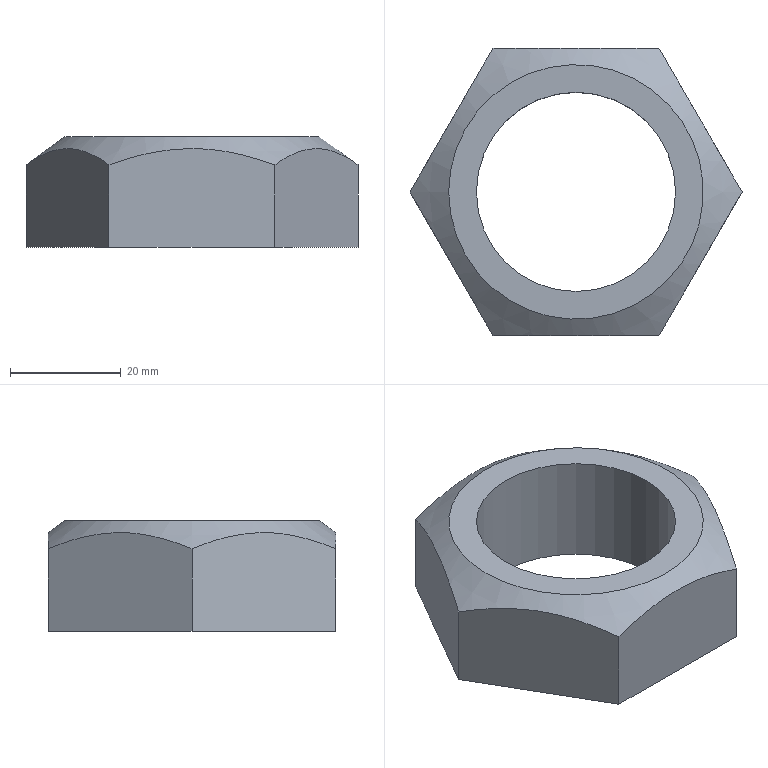Component | NX | A_PART_10 | 1 solid | 10 faces | box 60 x 51.96 x 20 mm | volume 25237 mm3 | plane 8 | cylinder 1 | cone 1 | commonest cylinder face diameters 36 x1
STEP:
#1=CARTESIAN_POINT('',(0.,0.,0.));
#2=DIRECTION('',(0.,0.,1.));
#3=DIRECTION('',(1.,0.,0.));
#4=AXIS2_PLACEMENT_3D('',#1,#2,#3);
#5=CARTESIAN_POINT('',(370.917,257.26,87.984));
#6=VERTEX_POINT('',#5);
#7=CARTESIAN_POINT('',(352.917,257.26,87.984));
#8=DIRECTION('',(0.,0.,1.));
#9=DIRECTION('',(1.,0.,0.));
#10=AXIS2_PLACEMENT_3D('',#7,#8,#9);
#11=CIRCLE('',#10,18.);
#12=CARTESIAN_POINT('',(352.917,257.26,87.984));
#13=DIRECTION('',(0.,0.,1.));
#14=DIRECTION('',(1.,0.,0.));
#15=AXIS2_PLACEMENT_3D('',#12,#13,#14);
#16=PLANE('',#15);
#17=CARTESIAN_POINT('',(0.,0.));
#18=DIRECTION('',(1.,0.));
#19=AXIS2_PLACEMENT_2D('',#17,#18);
#20=CIRCLE('',#19,18.);
#21=(GEOMETRIC_REPRESENTATION_CONTEXT(2)PARAMETRIC_REPRESENTATION_CONTEXT()REPRESENTATION_CONTEXT('',''));
#22=DEFINITIONAL_REPRESENTATION('',(#20),#21);
#23=PCURVE('',#16,#22);
#24=CARTESIAN_POINT('',(352.917,257.26,87.984));
#25=DIRECTION('',(0.,0.,-1.));
#26=DIRECTION('',(-1.,0.,0.));
#27=AXIS2_PLACEMENT_3D('',#24,#25,#26);
#28=CYLINDRICAL_SURFACE('',#27,18.);
#29=CARTESIAN_POINT('',(9.425,0.));
#30=DIRECTION('',(-1.,0.));
#31=VECTOR('',#30,1.);
#32=LINE('',#29,#31);
#33=(GEOMETRIC_REPRESENTATION_CONTEXT(2)PARAMETRIC_REPRESENTATION_CONTEXT()REPRESENTATION_CONTEXT('',''));
#34=DEFINITIONAL_REPRESENTATION('',(#32),#33);
#35=PCURVE('',#28,#34);
#36=SURFACE_CURVE('',#11,(#23,#35),.PCURVE_S1.);
#37=EDGE_CURVE('',#6,#6,#36,.T.);
#38=ORIENTED_EDGE('',*,*,#37,.F.);
#39=EDGE_LOOP('',(#38));
#40=FACE_BOUND('',#39,.T.);
#41=CARTESIAN_POINT('',(329.917,257.26,87.984));
#42=VERTEX_POINT('',#41);
#43=CARTESIAN_POINT('',(352.917,257.26,87.984));
#44=DIRECTION('',(0.,0.,-1.));
#45=DIRECTION('',(-1.,0.,0.));
#46=AXIS2_PLACEMENT_3D('',#43,#44,#45);
#47=CIRCLE('',#46,23.);
#48=CARTESIAN_POINT('',(-23.,0.));
#49=CARTESIAN_POINT('',(-23.,39.837));
#50=CARTESIAN_POINT('',(11.5,19.919));
#51=CARTESIAN_POINT('',(46.,0.));
#52=CARTESIAN_POINT('',(11.5,-19.919));
#53=CARTESIAN_POINT('',(-23.,-39.837));
#54=CARTESIAN_POINT('',(-23.,0.));
#55=(BOUNDED_CURVE()B_SPLINE_CURVE(2,(#48,#49,#50,#51,#52,#53,#54),.UNSPECIFIED.,.T.,.F.)B_SPLINE_CURVE_WITH_KNOTS((1,2,2,2,2,1),(-2.094,0.,2.094,4.189,6.283,8.378),.UNSPECIFIED.)CURVE()GEOMETRIC_REPRESENTATION_ITEM()RATIONAL_B_SPLINE_CURVE((1.,0.5,1.,0.5,1.,0.5,1.))REPRESENTATION_ITEM(''));
#56=(GEOMETRIC_REPRESENTATION_CONTEXT(2)PARAMETRIC_REPRESENTATION_CONTEXT()REPRESENTATION_CONTEXT('',''));
#57=DEFINITIONAL_REPRESENTATION('',(#55),#56);
#58=PCURVE('',#16,#57);
#59=CARTESIAN_POINT('',(352.917,257.26,87.984));
#60=DIRECTION('',(0.,0.,-1.));
#61=DIRECTION('',(-1.,0.,0.));
#62=AXIS2_PLACEMENT_3D('',#59,#60,#61);
#63=CONICAL_SURFACE('',#62,23.,0.9425);
#64=CARTESIAN_POINT('',(0.,0.));
#65=DIRECTION('',(1.,0.));
#66=VECTOR('',#65,1.);
#67=LINE('',#64,#66);
#68=(GEOMETRIC_REPRESENTATION_CONTEXT(2)PARAMETRIC_REPRESENTATION_CONTEXT()REPRESENTATION_CONTEXT('',''));
#69=DEFINITIONAL_REPRESENTATION('',(#67),#68);
#70=PCURVE('',#63,#69);
#71=SURFACE_CURVE('',#47,(#58,#70),.PCURVE_S1.);
#72=EDGE_CURVE('',#42,#42,#71,.T.);
#73=ORIENTED_EDGE('',*,*,#72,.F.);
#74=EDGE_LOOP('',(#73));
#75=FACE_BOUND('',#74,.T.);
#76=ADVANCED_FACE('',(#40,#75),#16,.T.);
#77=CARTESIAN_POINT('',(367.917,231.279,82.898));
#78=VERTEX_POINT('',#77);
#79=CARTESIAN_POINT('',(367.917,231.279,67.984));
#80=VERTEX_POINT('',#79);
#81=CARTESIAN_POINT('',(367.917,231.279,87.984));
#82=DIRECTION('',(0.,0.,-1.));
#83=VECTOR('',#82,1.);
#84=LINE('',#81,#83);
#85=CARTESIAN_POINT('',(337.917,231.279,87.984));
#86=DIRECTION('',(0.,1.,0.));
#87=DIRECTION('',(-1.,0.,0.));
#88=AXIS2_PLACEMENT_3D('',#85,#86,#87);
#89=PLANE('',#88);
#90=CARTESIAN_POINT('',(-30.,0.));
#91=DIRECTION('',(0.,-1.));
#92=VECTOR('',#91,1.);
#93=LINE('',#90,#92);
#94=(GEOMETRIC_REPRESENTATION_CONTEXT(2)PARAMETRIC_REPRESENTATION_CONTEXT()REPRESENTATION_CONTEXT('',''));
#95=DEFINITIONAL_REPRESENTATION('',(#93),#94);
#96=PCURVE('',#89,#95);
#97=CARTESIAN_POINT('',(367.917,231.279,87.984));
#98=DIRECTION('',(-0.866,0.5,0.));
#99=DIRECTION('',(-0.5,-0.866,0.));
#100=AXIS2_PLACEMENT_3D('',#97,#98,#99);
#101=PLANE('',#100);
#102=CARTESIAN_POINT('',(0.,0.));
#103=DIRECTION('',(0.,-1.));
#104=VECTOR('',#103,1.);
#105=LINE('',#102,#104);
#106=(GEOMETRIC_REPRESENTATION_CONTEXT(2)PARAMETRIC_REPRESENTATION_CONTEXT()REPRESENTATION_CONTEXT('',''));
#107=DEFINITIONAL_REPRESENTATION('',(#105),#106);
#108=PCURVE('',#101,#107);
#109=SURFACE_CURVE('',#84,(#96,#108),.PCURVE_S1.);
#110=EDGE_CURVE('',#78,#80,#109,.T.);
#111=ORIENTED_EDGE('',*,*,#110,.F.);
#112=CARTESIAN_POINT('',(337.917,231.279,82.898));
#113=VERTEX_POINT('',#112);
#114=CARTESIAN_POINT('',(367.917,231.279,82.898));
#115=CARTESIAN_POINT('',(365.498,231.279,83.776));
#116=CARTESIAN_POINT('',(363.045,231.279,84.51));
#117=CARTESIAN_POINT('',(358.03,231.279,85.536));
#118=CARTESIAN_POINT('',(355.435,231.279,85.821));
#119=CARTESIAN_POINT('',(347.77,231.279,85.813));
#120=CARTESIAN_POINT('',(342.723,231.279,84.644));
#121=CARTESIAN_POINT('',(337.917,231.279,82.898));
#122=B_SPLINE_CURVE_WITH_KNOTS('',3,(#114,#115,#116,#117,#118,#119,#120,#121),.UNSPECIFIED.,.F.,.F.,(4,2,2,4),(0.,0.25,0.5,1.),.UNSPECIFIED.);
#123=CARTESIAN_POINT('',(-30.,-5.086));
#124=CARTESIAN_POINT('',(-27.582,-4.207));
#125=CARTESIAN_POINT('',(-25.128,-3.474));
#126=CARTESIAN_POINT('',(-20.113,-2.448));
#127=CARTESIAN_POINT('',(-17.519,-2.163));
#128=CARTESIAN_POINT('',(-9.854,-2.171));
#129=CARTESIAN_POINT('',(-4.807,-3.34));
#130=CARTESIAN_POINT('',(0.,-5.086));
#131=B_SPLINE_CURVE_WITH_KNOTS('',3,(#123,#124,#125,#126,#127,#128,#129,#130),.UNSPECIFIED.,.F.,.F.,(4,2,2,4),(0.,0.25,0.5,1.),.UNSPECIFIED.);
#132=(GEOMETRIC_REPRESENTATION_CONTEXT(2)PARAMETRIC_REPRESENTATION_CONTEXT()REPRESENTATION_CONTEXT('',''));
#133=DEFINITIONAL_REPRESENTATION('',(#131),#132);
#134=PCURVE('',#89,#133);
#135=CARTESIAN_POINT('',(4.189,5.086));
#136=CARTESIAN_POINT('',(4.201,4.926));
#137=CARTESIAN_POINT('',(4.227,4.616));
#138=CARTESIAN_POINT('',(4.268,4.183));
#139=CARTESIAN_POINT('',(4.311,3.784));
#140=CARTESIAN_POINT('',(4.356,3.422));
#141=CARTESIAN_POINT('',(4.403,3.099));
#142=CARTESIAN_POINT('',(4.451,2.819));
#143=CARTESIAN_POINT('',(4.502,2.584));
#144=CARTESIAN_POINT('',(4.553,2.398));
#145=CARTESIAN_POINT('',(4.606,2.264));
#146=CARTESIAN_POINT('',(4.66,2.183));
#147=CARTESIAN_POINT('',(4.714,2.156));
#148=CARTESIAN_POINT('',(4.767,2.186));
#149=CARTESIAN_POINT('',(4.821,2.269));
#150=CARTESIAN_POINT('',(4.873,2.405));
#151=CARTESIAN_POINT('',(4.924,2.591));
#152=CARTESIAN_POINT('',(4.974,2.825));
#153=CARTESIAN_POINT('',(5.022,3.105));
#154=CARTESIAN_POINT('',(5.069,3.427));
#155=CARTESIAN_POINT('',(5.114,3.788));
#156=CARTESIAN_POINT('',(5.157,4.187));
#157=CARTESIAN_POINT('',(5.197,4.619));
#158=CARTESIAN_POINT('',(5.223,4.927));
#159=CARTESIAN_POINT('',(5.236,5.086));
#160=B_SPLINE_CURVE_WITH_KNOTS('',3,(#135,#136,#137,#138,#139,#140,#141,#142,#143,#144,#145,#146,#147,#148,#149,#150,#151,#152,#153,#154,#155,#156,#157,#158,#159),.UNSPECIFIED.,.F.,.F.,(4,1,1,1,1,1,1,1,1,1,1,1,1,1,1,1,1,1,1,1,1,1,4),(0.,0.04545,0.09091,0.1364,0.1818,0.2273,0.2727,0.3182,0.3636,0.4091,0.4545,0.5,0.5455,0.5909,0.6364,0.6818,0.7273,0.7727,0.8182,0.8636,0.9091,0.9545,1.),.QUASI_UNIFORM_KNOTS.);
#161=(GEOMETRIC_REPRESENTATION_CONTEXT(2)PARAMETRIC_REPRESENTATION_CONTEXT()REPRESENTATION_CONTEXT('',''));
#162=DEFINITIONAL_REPRESENTATION('',(#160),#161);
#163=PCURVE('',#63,#162);
#164=SURFACE_CURVE('',#122,(#134,#163),.PCURVE_S1.);
#165=EDGE_CURVE('',#78,#113,#164,.T.);
#166=ORIENTED_EDGE('',*,*,#165,.T.);
#167=CARTESIAN_POINT('',(337.917,231.279,67.984));
#168=VERTEX_POINT('',#167);
#169=CARTESIAN_POINT('',(337.917,231.279,87.984));
#170=DIRECTION('',(0.,0.,-1.));
#171=VECTOR('',#170,1.);
#172=LINE('',#169,#171);
#173=CARTESIAN_POINT('',(0.,0.));
#174=DIRECTION('',(0.,-1.));
#175=VECTOR('',#174,1.);
#176=LINE('',#173,#175);
#177=(GEOMETRIC_REPRESENTATION_CONTEXT(2)PARAMETRIC_REPRESENTATION_CONTEXT()REPRESENTATION_CONTEXT('',''));
#178=DEFINITIONAL_REPRESENTATION('',(#176),#177);
#179=PCURVE('',#89,#178);
#180=CARTESIAN_POINT('',(322.917,257.26,87.984));
#181=DIRECTION('',(0.866,0.5,0.));
#182=DIRECTION('',(-0.5,0.866,0.));
#183=AXIS2_PLACEMENT_3D('',#180,#181,#182);
#184=PLANE('',#183);
#185=CARTESIAN_POINT('',(-30.,0.));
#186=DIRECTION('',(0.,-1.));
#187=VECTOR('',#186,1.);
#188=LINE('',#185,#187);
#189=(GEOMETRIC_REPRESENTATION_CONTEXT(2)PARAMETRIC_REPRESENTATION_CONTEXT()REPRESENTATION_CONTEXT('',''));
#190=DEFINITIONAL_REPRESENTATION('',(#188),#189);
#191=PCURVE('',#184,#190);
#192=SURFACE_CURVE('',#172,(#179,#191),.PCURVE_S1.);
#193=EDGE_CURVE('',#113,#168,#192,.T.);
#194=ORIENTED_EDGE('',*,*,#193,.T.);
#195=CARTESIAN_POINT('',(337.917,231.279,67.984));
#196=DIRECTION('',(1.,-0.,0.));
#197=VECTOR('',#196,1.);
#198=LINE('',#195,#197);
#199=CARTESIAN_POINT('',(0.,-20.));
#200=DIRECTION('',(-1.,0.));
#201=VECTOR('',#200,1.);
#202=LINE('',#199,#201);
#203=(GEOMETRIC_REPRESENTATION_CONTEXT(2)PARAMETRIC_REPRESENTATION_CONTEXT()REPRESENTATION_CONTEXT('',''));
#204=DEFINITIONAL_REPRESENTATION('',(#202),#203);
#205=PCURVE('',#89,#204);
#206=CARTESIAN_POINT('',(352.917,257.26,67.984));
#207=DIRECTION('',(0.,0.,1.));
#208=DIRECTION('',(1.,0.,0.));
#209=AXIS2_PLACEMENT_3D('',#206,#207,#208);
#210=PLANE('',#209);
#211=CARTESIAN_POINT('',(-15.,-25.981));
#212=DIRECTION('',(1.,-0.));
#213=VECTOR('',#212,1.);
#214=LINE('',#211,#213);
#215=(GEOMETRIC_REPRESENTATION_CONTEXT(2)PARAMETRIC_REPRESENTATION_CONTEXT()REPRESENTATION_CONTEXT('',''));
#216=DEFINITIONAL_REPRESENTATION('',(#214),#215);
#217=PCURVE('',#210,#216);
#218=SURFACE_CURVE('',#198,(#205,#217),.PCURVE_S1.);
#219=EDGE_CURVE('',#168,#80,#218,.T.);
#220=ORIENTED_EDGE('',*,*,#219,.T.);
#221=EDGE_LOOP('',(#111,#166,#194,#220));
#222=FACE_BOUND('',#221,.T.);
#223=ADVANCED_FACE('',(#222),#89,.F.);
#224=CARTESIAN_POINT('',(382.917,257.26,82.898));
#225=VERTEX_POINT('',#224);
#226=CARTESIAN_POINT('',(382.917,257.26,67.984));
#227=VERTEX_POINT('',#226);
#228=CARTESIAN_POINT('',(382.917,257.26,87.984));
#229=DIRECTION('',(0.,0.,-1.));
#230=VECTOR('',#229,1.);
#231=LINE('',#228,#230);
#232=CARTESIAN_POINT('',(-30.,0.));
#233=DIRECTION('',(0.,-1.));
#234=VECTOR('',#233,1.);
#235=LINE('',#232,#234);
#236=(GEOMETRIC_REPRESENTATION_CONTEXT(2)PARAMETRIC_REPRESENTATION_CONTEXT()REPRESENTATION_CONTEXT('',''));
#237=DEFINITIONAL_REPRESENTATION('',(#235),#236);
#238=PCURVE('',#101,#237);
#239=CARTESIAN_POINT('',(382.917,257.26,87.984));
#240=DIRECTION('',(-0.866,-0.5,0.));
#241=DIRECTION('',(0.5,-0.866,0.));
#242=AXIS2_PLACEMENT_3D('',#239,#240,#241);
#243=PLANE('',#242);
#244=CARTESIAN_POINT('',(0.,0.));
#245=DIRECTION('',(0.,-1.));
#246=VECTOR('',#245,1.);
#247=LINE('',#244,#246);
#248=(GEOMETRIC_REPRESENTATION_CONTEXT(2)PARAMETRIC_REPRESENTATION_CONTEXT()REPRESENTATION_CONTEXT('',''));
#249=DEFINITIONAL_REPRESENTATION('',(#247),#248);
#250=PCURVE('',#243,#249);
#251=SURFACE_CURVE('',#231,(#238,#250),.PCURVE_S1.);
#252=EDGE_CURVE('',#225,#227,#251,.T.);
#253=ORIENTED_EDGE('',*,*,#252,.F.);
#254=CARTESIAN_POINT('',(382.917,257.26,82.898));
#255=CARTESIAN_POINT('',(380.496,253.067,84.657));
#256=CARTESIAN_POINT('',(378.023,248.783,85.808));
#257=CARTESIAN_POINT('',(374.164,242.099,85.823));
#258=CARTESIAN_POINT('',(372.869,239.857,85.538));
#259=CARTESIAN_POINT('',(370.361,235.513,84.515));
#260=CARTESIAN_POINT('',(369.131,233.382,83.78));
#261=CARTESIAN_POINT('',(367.917,231.279,82.898));
#262=B_SPLINE_CURVE_WITH_KNOTS('',3,(#254,#255,#256,#257,#258,#259,#260,#261),.UNSPECIFIED.,.F.,.F.,(4,2,2,4),(0.,0.5,0.75,1.),.UNSPECIFIED.);
#263=CARTESIAN_POINT('',(-30.,-5.086));
#264=CARTESIAN_POINT('',(-25.159,-3.327));
#265=CARTESIAN_POINT('',(-20.212,-2.175));
#266=CARTESIAN_POINT('',(-12.494,-2.161));
#267=CARTESIAN_POINT('',(-9.905,-2.445));
#268=CARTESIAN_POINT('',(-4.889,-3.469));
#269=CARTESIAN_POINT('',(-2.429,-4.204));
#270=CARTESIAN_POINT('',(0.,-5.086));
#271=B_SPLINE_CURVE_WITH_KNOTS('',3,(#263,#264,#265,#266,#267,#268,#269,#270),.UNSPECIFIED.,.F.,.F.,(4,2,2,4),(0.,0.5,0.75,1.),.UNSPECIFIED.);
#272=(GEOMETRIC_REPRESENTATION_CONTEXT(2)PARAMETRIC_REPRESENTATION_CONTEXT()REPRESENTATION_CONTEXT('',''));
#273=DEFINITIONAL_REPRESENTATION('',(#271),#272);
#274=PCURVE('',#101,#273);
#275=CARTESIAN_POINT('',(3.142,5.086));
#276=CARTESIAN_POINT('',(3.154,4.926));
#277=CARTESIAN_POINT('',(3.18,4.616));
#278=CARTESIAN_POINT('',(3.221,4.184));
#279=CARTESIAN_POINT('',(3.264,3.786));
#280=CARTESIAN_POINT('',(3.309,3.426));
#281=CARTESIAN_POINT('',(3.355,3.105));
#282=CARTESIAN_POINT('',(3.403,2.827));
#283=CARTESIAN_POINT('',(3.452,2.593));
#284=CARTESIAN_POINT('',(3.503,2.407));
#285=CARTESIAN_POINT('',(3.556,2.271));
#286=CARTESIAN_POINT('',(3.609,2.187));
#287=CARTESIAN_POINT('',(3.663,2.156));
#288=CARTESIAN_POINT('',(3.717,2.182));
#289=CARTESIAN_POINT('',(3.77,2.262));
#290=CARTESIAN_POINT('',(3.823,2.396));
#291=CARTESIAN_POINT('',(3.875,2.582));
#292=CARTESIAN_POINT('',(3.926,2.816));
#293=CARTESIAN_POINT('',(3.974,3.095));
#294=CARTESIAN_POINT('',(4.021,3.418));
#295=CARTESIAN_POINT('',(4.066,3.78));
#296=CARTESIAN_POINT('',(4.109,4.18));
#297=CARTESIAN_POINT('',(4.15,4.614));
#298=CARTESIAN_POINT('',(4.176,4.925));
#299=CARTESIAN_POINT('',(4.189,5.086));
#300=B_SPLINE_CURVE_WITH_KNOTS('',3,(#275,#276,#277,#278,#279,#280,#281,#282,#283,#284,#285,#286,#287,#288,#289,#290,#291,#292,#293,#294,#295,#296,#297,#298,#299),.UNSPECIFIED.,.F.,.F.,(4,1,1,1,1,1,1,1,1,1,1,1,1,1,1,1,1,1,1,1,1,1,4),(0.,0.04545,0.09091,0.1364,0.1818,0.2273,0.2727,0.3182,0.3636,0.4091,0.4545,0.5,0.5455,0.5909,0.6364,0.6818,0.7273,0.7727,0.8182,0.8636,0.9091,0.9545,1.),.QUASI_UNIFORM_KNOTS.);
#301=(GEOMETRIC_REPRESENTATION_CONTEXT(2)PARAMETRIC_REPRESENTATION_CONTEXT()REPRESENTATION_CONTEXT('',''));
#302=DEFINITIONAL_REPRESENTATION('',(#300),#301);
#303=PCURVE('',#63,#302);
#304=SURFACE_CURVE('',#262,(#274,#303),.PCURVE_S1.);
#305=EDGE_CURVE('',#225,#78,#304,.T.);
#306=ORIENTED_EDGE('',*,*,#305,.T.);
#307=ORIENTED_EDGE('',*,*,#110,.T.);
#308=CARTESIAN_POINT('',(367.917,231.279,67.984));
#309=DIRECTION('',(0.5,0.866,0.));
#310=VECTOR('',#309,1.);
#311=LINE('',#308,#310);
#312=CARTESIAN_POINT('',(0.,-20.));
#313=DIRECTION('',(-1.,0.));
#314=VECTOR('',#313,1.);
#315=LINE('',#312,#314);
#316=(GEOMETRIC_REPRESENTATION_CONTEXT(2)PARAMETRIC_REPRESENTATION_CONTEXT()REPRESENTATION_CONTEXT('',''));
#317=DEFINITIONAL_REPRESENTATION('',(#315),#316);
#318=PCURVE('',#101,#317);
#319=CARTESIAN_POINT('',(15.,-25.981));
#320=DIRECTION('',(0.5,0.866));
#321=VECTOR('',#320,1.);
#322=LINE('',#319,#321);
#323=(GEOMETRIC_REPRESENTATION_CONTEXT(2)PARAMETRIC_REPRESENTATION_CONTEXT()REPRESENTATION_CONTEXT('',''));
#324=DEFINITIONAL_REPRESENTATION('',(#322),#323);
#325=PCURVE('',#210,#324);
#326=SURFACE_CURVE('',#311,(#318,#325),.PCURVE_S1.);
#327=EDGE_CURVE('',#80,#227,#326,.T.);
#328=ORIENTED_EDGE('',*,*,#327,.T.);
#329=EDGE_LOOP('',(#253,#306,#307,#328));
#330=FACE_BOUND('',#329,.T.);
#331=ADVANCED_FACE('',(#330),#101,.F.);
#332=CARTESIAN_POINT('',(367.917,283.24,82.898));
#333=VERTEX_POINT('',#332);
#334=CARTESIAN_POINT('',(367.917,283.24,67.984));
#335=VERTEX_POINT('',#334);
#336=CARTESIAN_POINT('',(367.917,283.24,87.984));
#337=DIRECTION('',(0.,0.,-1.));
#338=VECTOR('',#337,1.);
#339=LINE('',#336,#338);
#340=CARTESIAN_POINT('',(-30.,0.));
#341=DIRECTION('',(0.,-1.));
#342=VECTOR('',#341,1.);
#343=LINE('',#340,#342);
#344=(GEOMETRIC_REPRESENTATION_CONTEXT(2)PARAMETRIC_REPRESENTATION_CONTEXT()REPRESENTATION_CONTEXT('',''));
#345=DEFINITIONAL_REPRESENTATION('',(#343),#344);
#346=PCURVE('',#243,#345);
#347=CARTESIAN_POINT('',(367.917,283.24,87.984));
#348=DIRECTION('',(-0.,-1.,0.));
#349=DIRECTION('',(1.,-0.,0.));
#350=AXIS2_PLACEMENT_3D('',#347,#348,#349);
#351=PLANE('',#350);
#352=CARTESIAN_POINT('',(0.,0.));
#353=DIRECTION('',(0.,-1.));
#354=VECTOR('',#353,1.);
#355=LINE('',#352,#354);
#356=(GEOMETRIC_REPRESENTATION_CONTEXT(2)PARAMETRIC_REPRESENTATION_CONTEXT()REPRESENTATION_CONTEXT('',''));
#357=DEFINITIONAL_REPRESENTATION('',(#355),#356);
#358=PCURVE('',#351,#357);
#359=SURFACE_CURVE('',#339,(#346,#358),.PCURVE_S1.);
#360=EDGE_CURVE('',#333,#335,#359,.T.);
#361=ORIENTED_EDGE('',*,*,#360,.F.);
#362=CARTESIAN_POINT('',(367.917,283.24,82.898));
#363=CARTESIAN_POINT('',(370.337,279.048,84.657));
#364=CARTESIAN_POINT('',(372.811,274.764,85.808));
#365=CARTESIAN_POINT('',(376.67,268.08,85.823));
#366=CARTESIAN_POINT('',(377.964,265.838,85.538));
#367=CARTESIAN_POINT('',(380.472,261.494,84.515));
#368=CARTESIAN_POINT('',(381.703,259.363,83.78));
#369=CARTESIAN_POINT('',(382.917,257.26,82.898));
#370=B_SPLINE_CURVE_WITH_KNOTS('',3,(#362,#363,#364,#365,#366,#367,#368,#369),.UNSPECIFIED.,.F.,.F.,(4,2,2,4),(0.,0.5,0.75,1.),.UNSPECIFIED.);
#371=CARTESIAN_POINT('',(-30.,-5.086));
#372=CARTESIAN_POINT('',(-25.159,-3.327));
#373=CARTESIAN_POINT('',(-20.212,-2.175));
#374=CARTESIAN_POINT('',(-12.494,-2.161));
#375=CARTESIAN_POINT('',(-9.905,-2.445));
#376=CARTESIAN_POINT('',(-4.889,-3.469));
#377=CARTESIAN_POINT('',(-2.429,-4.204));
#378=CARTESIAN_POINT('',(0.,-5.086));
#379=B_SPLINE_CURVE_WITH_KNOTS('',3,(#371,#372,#373,#374,#375,#376,#377,#378),.UNSPECIFIED.,.F.,.F.,(4,2,2,4),(0.,0.5,0.75,1.),.UNSPECIFIED.);
#380=(GEOMETRIC_REPRESENTATION_CONTEXT(2)PARAMETRIC_REPRESENTATION_CONTEXT()REPRESENTATION_CONTEXT('',''));
#381=DEFINITIONAL_REPRESENTATION('',(#379),#380);
#382=PCURVE('',#243,#381);
#383=CARTESIAN_POINT('',(2.094,5.086));
#384=CARTESIAN_POINT('',(2.107,4.926));
#385=CARTESIAN_POINT('',(2.133,4.616));
#386=CARTESIAN_POINT('',(2.174,4.184));
#387=CARTESIAN_POINT('',(2.217,3.786));
#388=CARTESIAN_POINT('',(2.261,3.426));
#389=CARTESIAN_POINT('',(2.308,3.105));
#390=CARTESIAN_POINT('',(2.356,2.827));
#391=CARTESIAN_POINT('',(2.405,2.593));
#392=CARTESIAN_POINT('',(2.456,2.407));
#393=CARTESIAN_POINT('',(2.508,2.271));
#394=CARTESIAN_POINT('',(2.562,2.187));
#395=CARTESIAN_POINT('',(2.615,2.156));
#396=CARTESIAN_POINT('',(2.669,2.182));
#397=CARTESIAN_POINT('',(2.723,2.262));
#398=CARTESIAN_POINT('',(2.776,2.396));
#399=CARTESIAN_POINT('',(2.828,2.582));
#400=CARTESIAN_POINT('',(2.878,2.816));
#401=CARTESIAN_POINT('',(2.927,3.095));
#402=CARTESIAN_POINT('',(2.974,3.418));
#403=CARTESIAN_POINT('',(3.019,3.78));
#404=CARTESIAN_POINT('',(3.062,4.18));
#405=CARTESIAN_POINT('',(3.103,4.614));
#406=CARTESIAN_POINT('',(3.129,4.925));
#407=CARTESIAN_POINT('',(3.142,5.086));
#408=B_SPLINE_CURVE_WITH_KNOTS('',3,(#383,#384,#385,#386,#387,#388,#389,#390,#391,#392,#393,#394,#395,#396,#397,#398,#399,#400,#401,#402,#403,#404,#405,#406,#407),.UNSPECIFIED.,.F.,.F.,(4,1,1,1,1,1,1,1,1,1,1,1,1,1,1,1,1,1,1,1,1,1,4),(0.,0.04545,0.09091,0.1364,0.1818,0.2273,0.2727,0.3182,0.3636,0.4091,0.4545,0.5,0.5455,0.5909,0.6364,0.6818,0.7273,0.7727,0.8182,0.8636,0.9091,0.9545,1.),.QUASI_UNIFORM_KNOTS.);
#409=(GEOMETRIC_REPRESENTATION_CONTEXT(2)PARAMETRIC_REPRESENTATION_CONTEXT()REPRESENTATION_CONTEXT('',''));
#410=DEFINITIONAL_REPRESENTATION('',(#408),#409);
#411=PCURVE('',#63,#410);
#412=SURFACE_CURVE('',#370,(#382,#411),.PCURVE_S1.);
#413=EDGE_CURVE('',#333,#225,#412,.T.);
#414=ORIENTED_EDGE('',*,*,#413,.T.);
#415=ORIENTED_EDGE('',*,*,#252,.T.);
#416=CARTESIAN_POINT('',(382.917,257.26,67.984));
#417=DIRECTION('',(-0.5,0.866,0.));
#418=VECTOR('',#417,1.);
#419=LINE('',#416,#418);
#420=CARTESIAN_POINT('',(0.,-20.));
#421=DIRECTION('',(-1.,0.));
#422=VECTOR('',#421,1.);
#423=LINE('',#420,#422);
#424=(GEOMETRIC_REPRESENTATION_CONTEXT(2)PARAMETRIC_REPRESENTATION_CONTEXT()REPRESENTATION_CONTEXT('',''));
#425=DEFINITIONAL_REPRESENTATION('',(#423),#424);
#426=PCURVE('',#243,#425);
#427=CARTESIAN_POINT('',(30.,0.));
#428=DIRECTION('',(-0.5,0.866));
#429=VECTOR('',#428,1.);
#430=LINE('',#427,#429);
#431=(GEOMETRIC_REPRESENTATION_CONTEXT(2)PARAMETRIC_REPRESENTATION_CONTEXT()REPRESENTATION_CONTEXT('',''));
#432=DEFINITIONAL_REPRESENTATION('',(#430),#431);
#433=PCURVE('',#210,#432);
#434=SURFACE_CURVE('',#419,(#426,#433),.PCURVE_S1.);
#435=EDGE_CURVE('',#227,#335,#434,.T.);
#436=ORIENTED_EDGE('',*,*,#435,.T.);
#437=EDGE_LOOP('',(#361,#414,#415,#436));
#438=FACE_BOUND('',#437,.T.);
#439=ADVANCED_FACE('',(#438),#243,.F.);
#440=CARTESIAN_POINT('',(337.917,283.24,82.898));
#441=VERTEX_POINT('',#440);
#442=CARTESIAN_POINT('',(337.917,283.24,67.984));
#443=VERTEX_POINT('',#442);
#444=CARTESIAN_POINT('',(337.917,283.24,87.984));
#445=DIRECTION('',(0.,0.,-1.));
#446=VECTOR('',#445,1.);
#447=LINE('',#444,#446);
#448=CARTESIAN_POINT('',(-30.,0.));
#449=DIRECTION('',(0.,-1.));
#450=VECTOR('',#449,1.);
#451=LINE('',#448,#450);
#452=(GEOMETRIC_REPRESENTATION_CONTEXT(2)PARAMETRIC_REPRESENTATION_CONTEXT()REPRESENTATION_CONTEXT('',''));
#453=DEFINITIONAL_REPRESENTATION('',(#451),#452);
#454=PCURVE('',#351,#453);
#455=CARTESIAN_POINT('',(337.917,283.24,87.984));
#456=DIRECTION('',(0.866,-0.5,0.));
#457=DIRECTION('',(0.5,0.866,0.));
#458=AXIS2_PLACEMENT_3D('',#455,#456,#457);
#459=PLANE('',#458);
#460=CARTESIAN_POINT('',(0.,0.));
#461=DIRECTION('',(0.,-1.));
#462=VECTOR('',#461,1.);
#463=LINE('',#460,#462);
#464=(GEOMETRIC_REPRESENTATION_CONTEXT(2)PARAMETRIC_REPRESENTATION_CONTEXT()REPRESENTATION_CONTEXT('',''));
#465=DEFINITIONAL_REPRESENTATION('',(#463),#464);
#466=PCURVE('',#459,#465);
#467=SURFACE_CURVE('',#447,(#454,#466),.PCURVE_S1.);
#468=EDGE_CURVE('',#441,#443,#467,.T.);
#469=ORIENTED_EDGE('',*,*,#468,.F.);
#470=CARTESIAN_POINT('',(337.917,283.24,82.898));
#471=CARTESIAN_POINT('',(342.723,283.24,84.644));
#472=CARTESIAN_POINT('',(347.77,283.24,85.813));
#473=CARTESIAN_POINT('',(355.435,283.24,85.821));
#474=CARTESIAN_POINT('',(358.03,283.24,85.536));
#475=CARTESIAN_POINT('',(363.045,283.24,84.51));
#476=CARTESIAN_POINT('',(365.498,283.24,83.776));
#477=CARTESIAN_POINT('',(367.917,283.24,82.898));
#478=B_SPLINE_CURVE_WITH_KNOTS('',3,(#470,#471,#472,#473,#474,#475,#476,#477),.UNSPECIFIED.,.F.,.F.,(4,2,2,4),(0.,0.5,0.75,1.),.UNSPECIFIED.);
#479=CARTESIAN_POINT('',(-30.,-5.086));
#480=CARTESIAN_POINT('',(-25.193,-3.34));
#481=CARTESIAN_POINT('',(-20.146,-2.171));
#482=CARTESIAN_POINT('',(-12.481,-2.163));
#483=CARTESIAN_POINT('',(-9.887,-2.448));
#484=CARTESIAN_POINT('',(-4.872,-3.474));
#485=CARTESIAN_POINT('',(-2.418,-4.207));
#486=CARTESIAN_POINT('',(0.,-5.086));
#487=B_SPLINE_CURVE_WITH_KNOTS('',3,(#479,#480,#481,#482,#483,#484,#485,#486),.UNSPECIFIED.,.F.,.F.,(4,2,2,4),(0.,0.5,0.75,1.),.UNSPECIFIED.);
#488=(GEOMETRIC_REPRESENTATION_CONTEXT(2)PARAMETRIC_REPRESENTATION_CONTEXT()REPRESENTATION_CONTEXT('',''));
#489=DEFINITIONAL_REPRESENTATION('',(#487),#488);
#490=PCURVE('',#351,#489);
#491=CARTESIAN_POINT('',(1.047,5.086));
#492=CARTESIAN_POINT('',(1.06,4.927));
#493=CARTESIAN_POINT('',(1.086,4.619));
#494=CARTESIAN_POINT('',(1.127,4.187));
#495=CARTESIAN_POINT('',(1.169,3.788));
#496=CARTESIAN_POINT('',(1.214,3.427));
#497=CARTESIAN_POINT('',(1.261,3.105));
#498=CARTESIAN_POINT('',(1.309,2.825));
#499=CARTESIAN_POINT('',(1.359,2.591));
#500=CARTESIAN_POINT('',(1.41,2.405));
#501=CARTESIAN_POINT('',(1.463,2.269));
#502=CARTESIAN_POINT('',(1.516,2.186));
#503=CARTESIAN_POINT('',(1.569,2.156));
#504=CARTESIAN_POINT('',(1.623,2.183));
#505=CARTESIAN_POINT('',(1.677,2.264));
#506=CARTESIAN_POINT('',(1.73,2.398));
#507=CARTESIAN_POINT('',(1.782,2.584));
#508=CARTESIAN_POINT('',(1.832,2.819));
#509=CARTESIAN_POINT('',(1.88,3.099));
#510=CARTESIAN_POINT('',(1.927,3.422));
#511=CARTESIAN_POINT('',(1.972,3.784));
#512=CARTESIAN_POINT('',(2.015,4.183));
#513=CARTESIAN_POINT('',(2.056,4.616));
#514=CARTESIAN_POINT('',(2.082,4.926));
#515=CARTESIAN_POINT('',(2.094,5.086));
#516=B_SPLINE_CURVE_WITH_KNOTS('',3,(#491,#492,#493,#494,#495,#496,#497,#498,#499,#500,#501,#502,#503,#504,#505,#506,#507,#508,#509,#510,#511,#512,#513,#514,#515),.UNSPECIFIED.,.F.,.F.,(4,1,1,1,1,1,1,1,1,1,1,1,1,1,1,1,1,1,1,1,1,1,4),(0.,0.04545,0.09091,0.1364,0.1818,0.2273,0.2727,0.3182,0.3636,0.4091,0.4545,0.5,0.5455,0.5909,0.6364,0.6818,0.7273,0.7727,0.8182,0.8636,0.9091,0.9545,1.),.QUASI_UNIFORM_KNOTS.);
#517=(GEOMETRIC_REPRESENTATION_CONTEXT(2)PARAMETRIC_REPRESENTATION_CONTEXT()REPRESENTATION_CONTEXT('',''));
#518=DEFINITIONAL_REPRESENTATION('',(#516),#517);
#519=PCURVE('',#63,#518);
#520=SURFACE_CURVE('',#478,(#490,#519),.PCURVE_S1.);
#521=EDGE_CURVE('',#441,#333,#520,.T.);
#522=ORIENTED_EDGE('',*,*,#521,.T.);
#523=ORIENTED_EDGE('',*,*,#360,.T.);
#524=CARTESIAN_POINT('',(367.917,283.24,67.984));
#525=DIRECTION('',(-1.,0.,0.));
#526=VECTOR('',#525,1.);
#527=LINE('',#524,#526);
#528=CARTESIAN_POINT('',(0.,-20.));
#529=DIRECTION('',(-1.,0.));
#530=VECTOR('',#529,1.);
#531=LINE('',#528,#530);
#532=(GEOMETRIC_REPRESENTATION_CONTEXT(2)PARAMETRIC_REPRESENTATION_CONTEXT()REPRESENTATION_CONTEXT('',''));
#533=DEFINITIONAL_REPRESENTATION('',(#531),#532);
#534=PCURVE('',#351,#533);
#535=CARTESIAN_POINT('',(15.,25.981));
#536=DIRECTION('',(-1.,0.));
#537=VECTOR('',#536,1.);
#538=LINE('',#535,#537);
#539=(GEOMETRIC_REPRESENTATION_CONTEXT(2)PARAMETRIC_REPRESENTATION_CONTEXT()REPRESENTATION_CONTEXT('',''));
#540=DEFINITIONAL_REPRESENTATION('',(#538),#539);
#541=PCURVE('',#210,#540);
#542=SURFACE_CURVE('',#527,(#534,#541),.PCURVE_S1.);
#543=EDGE_CURVE('',#335,#443,#542,.T.);
#544=ORIENTED_EDGE('',*,*,#543,.T.);
#545=EDGE_LOOP('',(#469,#522,#523,#544));
#546=FACE_BOUND('',#545,.T.);
#547=ADVANCED_FACE('',(#546),#351,.F.);
#548=CARTESIAN_POINT('',(322.917,257.26,82.898));
#549=VERTEX_POINT('',#548);
#550=CARTESIAN_POINT('',(322.917,257.26,67.984));
#551=VERTEX_POINT('',#550);
#552=CARTESIAN_POINT('',(322.917,257.26,87.984));
#553=DIRECTION('',(0.,0.,-1.));
#554=VECTOR('',#553,1.);
#555=LINE('',#552,#554);
#556=CARTESIAN_POINT('',(-30.,0.));
#557=DIRECTION('',(0.,-1.));
#558=VECTOR('',#557,1.);
#559=LINE('',#556,#558);
#560=(GEOMETRIC_REPRESENTATION_CONTEXT(2)PARAMETRIC_REPRESENTATION_CONTEXT()REPRESENTATION_CONTEXT('',''));
#561=DEFINITIONAL_REPRESENTATION('',(#559),#560);
#562=PCURVE('',#459,#561);
#563=CARTESIAN_POINT('',(0.,0.));
#564=DIRECTION('',(0.,-1.));
#565=VECTOR('',#564,1.);
#566=LINE('',#563,#565);
#567=(GEOMETRIC_REPRESENTATION_CONTEXT(2)PARAMETRIC_REPRESENTATION_CONTEXT()REPRESENTATION_CONTEXT('',''));
#568=DEFINITIONAL_REPRESENTATION('',(#566),#567);
#569=PCURVE('',#184,#568);
#570=SURFACE_CURVE('',#555,(#562,#569),.PCURVE_S1.);
#571=EDGE_CURVE('',#549,#551,#570,.T.);
#572=ORIENTED_EDGE('',*,*,#571,.F.);
#573=CARTESIAN_POINT('',(322.917,257.26,82.898));
#574=CARTESIAN_POINT('',(325.337,261.452,84.657));
#575=CARTESIAN_POINT('',(327.811,265.736,85.808));
#576=CARTESIAN_POINT('',(331.67,272.42,85.823));
#577=CARTESIAN_POINT('',(332.964,274.662,85.538));
#578=CARTESIAN_POINT('',(335.472,279.006,84.515));
#579=CARTESIAN_POINT('',(336.703,281.137,83.78));
#580=CARTESIAN_POINT('',(337.917,283.24,82.898));
#581=B_SPLINE_CURVE_WITH_KNOTS('',3,(#573,#574,#575,#576,#577,#578,#579,#580),.UNSPECIFIED.,.F.,.F.,(4,2,2,4),(0.,0.5,0.75,1.),.UNSPECIFIED.);
#582=CARTESIAN_POINT('',(-30.,-5.086));
#583=CARTESIAN_POINT('',(-25.159,-3.327));
#584=CARTESIAN_POINT('',(-20.212,-2.175));
#585=CARTESIAN_POINT('',(-12.494,-2.161));
#586=CARTESIAN_POINT('',(-9.905,-2.445));
#587=CARTESIAN_POINT('',(-4.889,-3.469));
#588=CARTESIAN_POINT('',(-2.429,-4.204));
#589=CARTESIAN_POINT('',(0.,-5.086));
#590=B_SPLINE_CURVE_WITH_KNOTS('',3,(#582,#583,#584,#585,#586,#587,#588,#589),.UNSPECIFIED.,.F.,.F.,(4,2,2,4),(0.,0.5,0.75,1.),.UNSPECIFIED.);
#591=(GEOMETRIC_REPRESENTATION_CONTEXT(2)PARAMETRIC_REPRESENTATION_CONTEXT()REPRESENTATION_CONTEXT('',''));
#592=DEFINITIONAL_REPRESENTATION('',(#590),#591);
#593=PCURVE('',#459,#592);
#594=CARTESIAN_POINT('',(0.,5.086));
#595=CARTESIAN_POINT('',(0.0127,4.926));
#596=CARTESIAN_POINT('',(0.03873,4.616));
#597=CARTESIAN_POINT('',(0.07961,4.184));
#598=CARTESIAN_POINT('',(0.1223,3.786));
#599=CARTESIAN_POINT('',(0.1669,3.426));
#600=CARTESIAN_POINT('',(0.2133,3.105));
#601=CARTESIAN_POINT('',(0.2613,2.827));
#602=CARTESIAN_POINT('',(0.3109,2.593));
#603=CARTESIAN_POINT('',(0.3618,2.407));
#604=CARTESIAN_POINT('',(0.414,2.271));
#605=CARTESIAN_POINT('',(0.4671,2.187));
#606=CARTESIAN_POINT('',(0.521,2.156));
#607=CARTESIAN_POINT('',(0.5751,2.182));
#608=CARTESIAN_POINT('',(0.6289,2.262));
#609=CARTESIAN_POINT('',(0.6819,2.396));
#610=CARTESIAN_POINT('',(0.7337,2.582));
#611=CARTESIAN_POINT('',(0.7841,2.816));
#612=CARTESIAN_POINT('',(0.8326,3.095));
#613=CARTESIAN_POINT('',(0.8794,3.418));
#614=CARTESIAN_POINT('',(0.9243,3.78));
#615=CARTESIAN_POINT('',(0.9673,4.18));
#616=CARTESIAN_POINT('',(1.008,4.614));
#617=CARTESIAN_POINT('',(1.034,4.925));
#618=CARTESIAN_POINT('',(1.047,5.086));
#619=B_SPLINE_CURVE_WITH_KNOTS('',3,(#594,#595,#596,#597,#598,#599,#600,#601,#602,#603,#604,#605,#606,#607,#608,#609,#610,#611,#612,#613,#614,#615,#616,#617,#618),.UNSPECIFIED.,.F.,.F.,(4,1,1,1,1,1,1,1,1,1,1,1,1,1,1,1,1,1,1,1,1,1,4),(0.,0.04545,0.09091,0.1364,0.1818,0.2273,0.2727,0.3182,0.3636,0.4091,0.4545,0.5,0.5455,0.5909,0.6364,0.6818,0.7273,0.7727,0.8182,0.8636,0.9091,0.9545,1.),.QUASI_UNIFORM_KNOTS.);
#620=(GEOMETRIC_REPRESENTATION_CONTEXT(2)PARAMETRIC_REPRESENTATION_CONTEXT()REPRESENTATION_CONTEXT('',''));
#621=DEFINITIONAL_REPRESENTATION('',(#619),#620);
#622=PCURVE('',#63,#621);
#623=SURFACE_CURVE('',#581,(#593,#622),.PCURVE_S1.);
#624=EDGE_CURVE('',#549,#441,#623,.T.);
#625=ORIENTED_EDGE('',*,*,#624,.T.);
#626=ORIENTED_EDGE('',*,*,#468,.T.);
#627=CARTESIAN_POINT('',(337.917,283.24,67.984));
#628=DIRECTION('',(-0.5,-0.866,0.));
#629=VECTOR('',#628,1.);
#630=LINE('',#627,#629);
#631=CARTESIAN_POINT('',(0.,-20.));
#632=DIRECTION('',(-1.,0.));
#633=VECTOR('',#632,1.);
#634=LINE('',#631,#633);
#635=(GEOMETRIC_REPRESENTATION_CONTEXT(2)PARAMETRIC_REPRESENTATION_CONTEXT()REPRESENTATION_CONTEXT('',''));
#636=DEFINITIONAL_REPRESENTATION('',(#634),#635);
#637=PCURVE('',#459,#636);
#638=CARTESIAN_POINT('',(-15.,25.981));
#639=DIRECTION('',(-0.5,-0.866));
#640=VECTOR('',#639,1.);
#641=LINE('',#638,#640);
#642=(GEOMETRIC_REPRESENTATION_CONTEXT(2)PARAMETRIC_REPRESENTATION_CONTEXT()REPRESENTATION_CONTEXT('',''));
#643=DEFINITIONAL_REPRESENTATION('',(#641),#642);
#644=PCURVE('',#210,#643);
#645=SURFACE_CURVE('',#630,(#637,#644),.PCURVE_S1.);
#646=EDGE_CURVE('',#443,#551,#645,.T.);
#647=ORIENTED_EDGE('',*,*,#646,.T.);
#648=EDGE_LOOP('',(#572,#625,#626,#647));
#649=FACE_BOUND('',#648,.T.);
#650=ADVANCED_FACE('',(#649),#459,.F.);
#651=ORIENTED_EDGE('',*,*,#193,.F.);
#652=CARTESIAN_POINT('',(337.917,231.279,82.898));
#653=CARTESIAN_POINT('',(335.496,235.471,84.657));
#654=CARTESIAN_POINT('',(333.023,239.755,85.808));
#655=CARTESIAN_POINT('',(329.164,246.439,85.823));
#656=CARTESIAN_POINT('',(327.869,248.681,85.538));
#657=CARTESIAN_POINT('',(325.361,253.026,84.515));
#658=CARTESIAN_POINT('',(324.131,255.156,83.78));
#659=CARTESIAN_POINT('',(322.917,257.26,82.898));
#660=B_SPLINE_CURVE_WITH_KNOTS('',3,(#652,#653,#654,#655,#656,#657,#658,#659),.UNSPECIFIED.,.F.,.F.,(4,2,2,4),(0.,0.5,0.75,1.),.UNSPECIFIED.);
#661=CARTESIAN_POINT('',(-30.,-5.086));
#662=CARTESIAN_POINT('',(-25.159,-3.327));
#663=CARTESIAN_POINT('',(-20.212,-2.175));
#664=CARTESIAN_POINT('',(-12.494,-2.161));
#665=CARTESIAN_POINT('',(-9.905,-2.445));
#666=CARTESIAN_POINT('',(-4.889,-3.469));
#667=CARTESIAN_POINT('',(-2.429,-4.204));
#668=CARTESIAN_POINT('',(0.,-5.086));
#669=B_SPLINE_CURVE_WITH_KNOTS('',3,(#661,#662,#663,#664,#665,#666,#667,#668),.UNSPECIFIED.,.F.,.F.,(4,2,2,4),(0.,0.5,0.75,1.),.UNSPECIFIED.);
#670=(GEOMETRIC_REPRESENTATION_CONTEXT(2)PARAMETRIC_REPRESENTATION_CONTEXT()REPRESENTATION_CONTEXT('',''));
#671=DEFINITIONAL_REPRESENTATION('',(#669),#670);
#672=PCURVE('',#184,#671);
#673=CARTESIAN_POINT('',(5.236,5.086));
#674=CARTESIAN_POINT('',(5.249,4.926));
#675=CARTESIAN_POINT('',(5.275,4.616));
#676=CARTESIAN_POINT('',(5.316,4.184));
#677=CARTESIAN_POINT('',(5.358,3.786));
#678=CARTESIAN_POINT('',(5.403,3.426));
#679=CARTESIAN_POINT('',(5.449,3.105));
#680=CARTESIAN_POINT('',(5.497,2.827));
#681=CARTESIAN_POINT('',(5.547,2.593));
#682=CARTESIAN_POINT('',(5.598,2.407));
#683=CARTESIAN_POINT('',(5.65,2.271));
#684=CARTESIAN_POINT('',(5.703,2.187));
#685=CARTESIAN_POINT('',(5.757,2.156));
#686=CARTESIAN_POINT('',(5.811,2.182));
#687=CARTESIAN_POINT('',(5.865,2.262));
#688=CARTESIAN_POINT('',(5.918,2.396));
#689=CARTESIAN_POINT('',(5.97,2.582));
#690=CARTESIAN_POINT('',(6.02,2.816));
#691=CARTESIAN_POINT('',(6.069,3.095));
#692=CARTESIAN_POINT('',(6.115,3.418));
#693=CARTESIAN_POINT('',(6.16,3.78));
#694=CARTESIAN_POINT('',(6.203,4.18));
#695=CARTESIAN_POINT('',(6.244,4.614));
#696=CARTESIAN_POINT('',(6.27,4.925));
#697=CARTESIAN_POINT('',(6.283,5.086));
#698=B_SPLINE_CURVE_WITH_KNOTS('',3,(#673,#674,#675,#676,#677,#678,#679,#680,#681,#682,#683,#684,#685,#686,#687,#688,#689,#690,#691,#692,#693,#694,#695,#696,#697),.UNSPECIFIED.,.F.,.F.,(4,1,1,1,1,1,1,1,1,1,1,1,1,1,1,1,1,1,1,1,1,1,4),(0.,0.04545,0.09091,0.1364,0.1818,0.2273,0.2727,0.3182,0.3636,0.4091,0.4545,0.5,0.5455,0.5909,0.6364,0.6818,0.7273,0.7727,0.8182,0.8636,0.9091,0.9545,1.),.QUASI_UNIFORM_KNOTS.);
#699=(GEOMETRIC_REPRESENTATION_CONTEXT(2)PARAMETRIC_REPRESENTATION_CONTEXT()REPRESENTATION_CONTEXT('',''));
#700=DEFINITIONAL_REPRESENTATION('',(#698),#699);
#701=PCURVE('',#63,#700);
#702=SURFACE_CURVE('',#660,(#672,#701),.PCURVE_S1.);
#703=EDGE_CURVE('',#113,#549,#702,.T.);
#704=ORIENTED_EDGE('',*,*,#703,.T.);
#705=ORIENTED_EDGE('',*,*,#571,.T.);
#706=CARTESIAN_POINT('',(322.917,257.26,67.984));
#707=DIRECTION('',(0.5,-0.866,0.));
#708=VECTOR('',#707,1.);
#709=LINE('',#706,#708);
#710=CARTESIAN_POINT('',(0.,-20.));
#711=DIRECTION('',(-1.,0.));
#712=VECTOR('',#711,1.);
#713=LINE('',#710,#712);
#714=(GEOMETRIC_REPRESENTATION_CONTEXT(2)PARAMETRIC_REPRESENTATION_CONTEXT()REPRESENTATION_CONTEXT('',''));
#715=DEFINITIONAL_REPRESENTATION('',(#713),#714);
#716=PCURVE('',#184,#715);
#717=CARTESIAN_POINT('',(-30.,0.));
#718=DIRECTION('',(0.5,-0.866));
#719=VECTOR('',#718,1.);
#720=LINE('',#717,#719);
#721=(GEOMETRIC_REPRESENTATION_CONTEXT(2)PARAMETRIC_REPRESENTATION_CONTEXT()REPRESENTATION_CONTEXT('',''));
#722=DEFINITIONAL_REPRESENTATION('',(#720),#721);
#723=PCURVE('',#210,#722);
#724=SURFACE_CURVE('',#709,(#716,#723),.PCURVE_S1.);
#725=EDGE_CURVE('',#551,#168,#724,.T.);
#726=ORIENTED_EDGE('',*,*,#725,.T.);
#727=EDGE_LOOP('',(#651,#704,#705,#726));
#728=FACE_BOUND('',#727,.T.);
#729=ADVANCED_FACE('',(#728),#184,.F.);
#730=ORIENTED_EDGE('',*,*,#37,.F.);
#731=CARTESIAN_POINT('',(370.917,257.26,67.984));
#732=VERTEX_POINT('',#731);
#733=CARTESIAN_POINT('',(370.917,257.26,87.984));
#734=CARTESIAN_POINT('',(370.917,257.26,67.984));
#735=B_SPLINE_CURVE_WITH_KNOTS('',1,(#733,#734),.UNSPECIFIED.,.F.,.F.,(2,2),(0.,20.),.PIECEWISE_BEZIER_KNOTS.);
#736=CARTESIAN_POINT('',(9.425,0.));
#737=DIRECTION('',(0.,1.));
#738=VECTOR('',#737,1.);
#739=LINE('',#736,#738);
#740=(GEOMETRIC_REPRESENTATION_CONTEXT(2)PARAMETRIC_REPRESENTATION_CONTEXT()REPRESENTATION_CONTEXT('',''));
#741=DEFINITIONAL_REPRESENTATION('',(#739),#740);
#742=PCURVE('',#28,#741);
#743=CARTESIAN_POINT('',(3.142,0.));
#744=DIRECTION('',(0.,1.));
#745=VECTOR('',#744,1.);
#746=LINE('',#743,#745);
#747=(GEOMETRIC_REPRESENTATION_CONTEXT(2)PARAMETRIC_REPRESENTATION_CONTEXT()REPRESENTATION_CONTEXT('',''));
#748=DEFINITIONAL_REPRESENTATION('',(#746),#747);
#749=PCURVE('',#28,#748);
#750=SEAM_CURVE('',#735,(#742,#749),.PCURVE_S1.);
#751=EDGE_CURVE('',#6,#732,#750,.T.);
#752=ORIENTED_EDGE('',*,*,#751,.T.);
#753=CARTESIAN_POINT('',(352.917,257.26,67.984));
#754=DIRECTION('',(0.,0.,1.));
#755=DIRECTION('',(1.,0.,0.));
#756=AXIS2_PLACEMENT_3D('',#753,#754,#755);
#757=CIRCLE('',#756,18.);
#758=CARTESIAN_POINT('',(9.425,20.));
#759=DIRECTION('',(-1.,0.));
#760=VECTOR('',#759,1.);
#761=LINE('',#758,#760);
#762=(GEOMETRIC_REPRESENTATION_CONTEXT(2)PARAMETRIC_REPRESENTATION_CONTEXT()REPRESENTATION_CONTEXT('',''));
#763=DEFINITIONAL_REPRESENTATION('',(#761),#762);
#764=PCURVE('',#28,#763);
#765=CARTESIAN_POINT('',(0.,0.));
#766=DIRECTION('',(1.,0.));
#767=AXIS2_PLACEMENT_2D('',#765,#766);
#768=CIRCLE('',#767,18.);
#769=(GEOMETRIC_REPRESENTATION_CONTEXT(2)PARAMETRIC_REPRESENTATION_CONTEXT()REPRESENTATION_CONTEXT('',''));
#770=DEFINITIONAL_REPRESENTATION('',(#768),#769);
#771=PCURVE('',#210,#770);
#772=SURFACE_CURVE('',#757,(#764,#771),.PCURVE_S1.);
#773=EDGE_CURVE('',#732,#732,#772,.T.);
#774=ORIENTED_EDGE('',*,*,#773,.T.);
#775=ORIENTED_EDGE('',*,*,#751,.F.);
#776=EDGE_LOOP('',(#730,#752,#774,#775));
#777=FACE_BOUND('',#776,.F.);
#778=ADVANCED_FACE('',(#777),#28,.F.);
#779=ORIENTED_EDGE('',*,*,#219,.F.);
#780=ORIENTED_EDGE('',*,*,#725,.F.);
#781=ORIENTED_EDGE('',*,*,#646,.F.);
#782=ORIENTED_EDGE('',*,*,#543,.F.);
#783=ORIENTED_EDGE('',*,*,#435,.F.);
#784=ORIENTED_EDGE('',*,*,#327,.F.);
#785=EDGE_LOOP('',(#779,#780,#781,#782,#783,#784));
#786=FACE_BOUND('',#785,.T.);
#787=ORIENTED_EDGE('',*,*,#773,.T.);
#788=EDGE_LOOP('',(#787));
#789=FACE_BOUND('',#788,.T.);
#790=ADVANCED_FACE('',(#786,#789),#210,.F.);
#791=ORIENTED_EDGE('',*,*,#72,.T.);
#792=CARTESIAN_POINT('',(329.917,257.26,87.984));
#793=CARTESIAN_POINT('',(322.917,257.26,82.898));
#794=B_SPLINE_CURVE_WITH_KNOTS('',1,(#792,#793),.UNSPECIFIED.,.F.,.F.,(2,2),(0.,8.652),.PIECEWISE_BEZIER_KNOTS.);
#795=CARTESIAN_POINT('',(6.283,0.));
#796=DIRECTION('',(0.,1.));
#797=VECTOR('',#796,1.);
#798=LINE('',#795,#797);
#799=(GEOMETRIC_REPRESENTATION_CONTEXT(2)PARAMETRIC_REPRESENTATION_CONTEXT()REPRESENTATION_CONTEXT('',''));
#800=DEFINITIONAL_REPRESENTATION('',(#798),#799);
#801=PCURVE('',#63,#800);
#802=CARTESIAN_POINT('',(0.,0.));
#803=DIRECTION('',(0.,1.));
#804=VECTOR('',#803,1.);
#805=LINE('',#802,#804);
#806=(GEOMETRIC_REPRESENTATION_CONTEXT(2)PARAMETRIC_REPRESENTATION_CONTEXT()REPRESENTATION_CONTEXT('',''));
#807=DEFINITIONAL_REPRESENTATION('',(#805),#806);
#808=PCURVE('',#63,#807);
#809=SEAM_CURVE('',#794,(#801,#808),.PCURVE_S1.);
#810=EDGE_CURVE('',#42,#549,#809,.T.);
#811=ORIENTED_EDGE('',*,*,#810,.T.);
#812=ORIENTED_EDGE('',*,*,#703,.F.);
#813=ORIENTED_EDGE('',*,*,#165,.F.);
#814=ORIENTED_EDGE('',*,*,#305,.F.);
#815=ORIENTED_EDGE('',*,*,#413,.F.);
#816=ORIENTED_EDGE('',*,*,#521,.F.);
#817=ORIENTED_EDGE('',*,*,#624,.F.);
#818=ORIENTED_EDGE('',*,*,#810,.F.);
#819=EDGE_LOOP('',(#791,#811,#812,#813,#814,#815,#816,#817,#818));
#820=FACE_BOUND('',#819,.T.);
#821=ADVANCED_FACE('',(#820),#63,.T.);
#822=CLOSED_SHELL('',(#76,#223,#331,#439,#547,#650,#729,#778,#790,#821));
#823=MANIFOLD_SOLID_BREP('',#822);
#824=(LENGTH_UNIT()NAMED_UNIT(*)SI_UNIT(.MILLI.,.METRE.));
#825=UNCERTAINTY_MEASURE_WITH_UNIT(LENGTH_MEASURE(0.002),#824,'','');
#826=(NAMED_UNIT(*)PLANE_ANGLE_UNIT()SI_UNIT($,.RADIAN.));
#827=(NAMED_UNIT(*)SI_UNIT($,.STERADIAN.)SOLID_ANGLE_UNIT());
#828=(GEOMETRIC_REPRESENTATION_CONTEXT(3)GLOBAL_UNCERTAINTY_ASSIGNED_CONTEXT((#825))GLOBAL_UNIT_ASSIGNED_CONTEXT((#824,#826,#827))REPRESENTATION_CONTEXT('',''));
#829=ADVANCED_BREP_SHAPE_REPRESENTATION('',(#4,#823),#828);